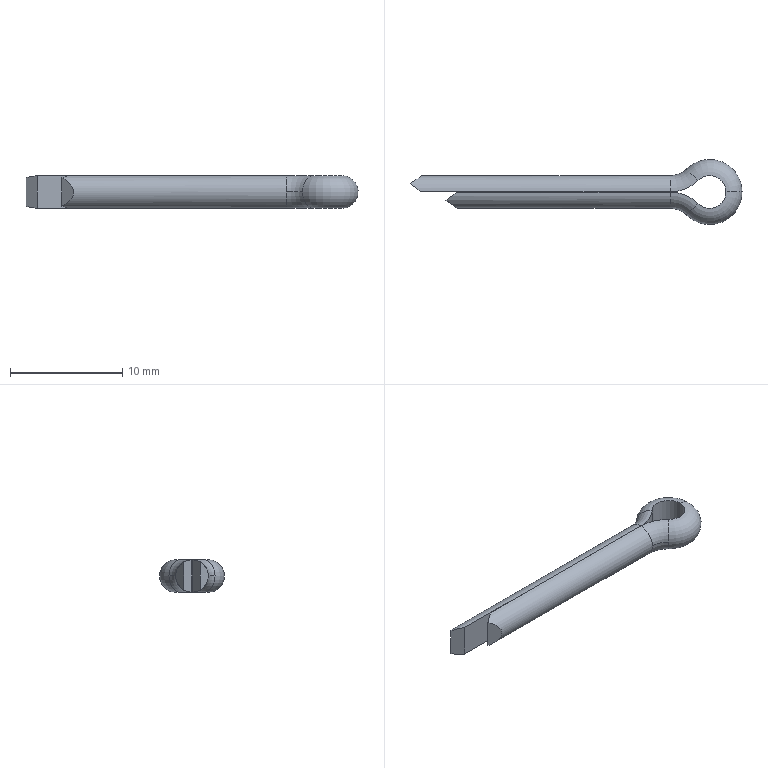Component | NX | GB_T_91_2000_COTTERPIN_3_2X20 | 1 solid | 17 faces | volume 185 mm3 | torus 6 | plane 6 | cylinder 5 | commonest cylinder face diameters 2.9 x2 6.978 x2 2.92 x1